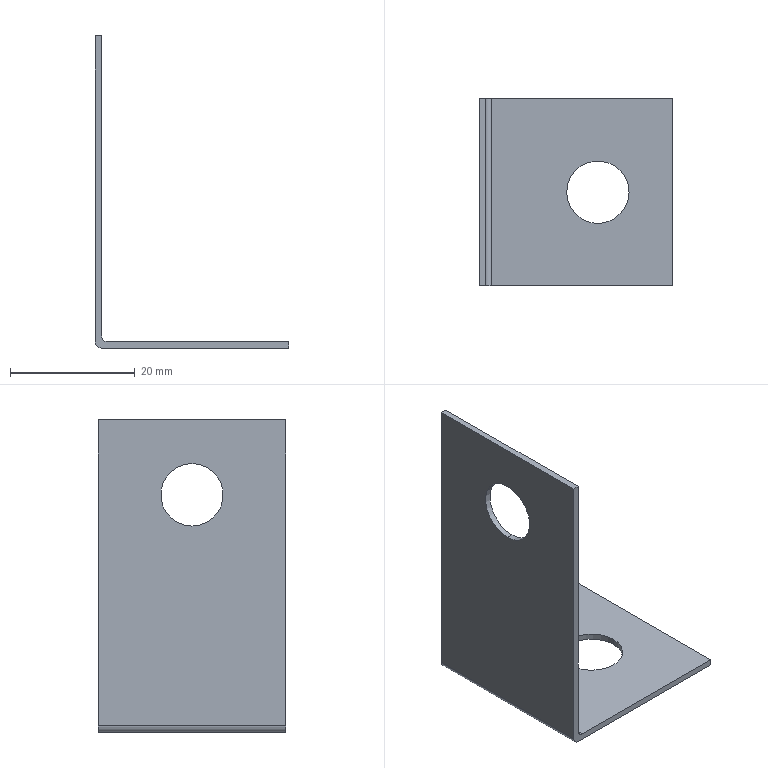Component | SolidWorks | ThreadedConnectionPlate-1 | 1 solid | 14 faces | box 31 x 30 x 50 mm | volume 2243 mm3 | plane 8 | cylinder 6 | commonest cylinder face diameters 10 x4 2 x2
build123d program:
from build123d import *

# Parameters (mm, degrees)
SKETCH1_W           = 30
SKETCH1_H           = 30
BOSS_EXTRUDE1_DEPTH = 1
SKETCH2_W           = 50
SKETCH2_H           = 30
BOSS_EXTRUDE2_DEPTH = 1
FILLET1_R           = 1
SKETCH3_R           = 5
CUT_EXTRUDE1_DEPTH  = 1
SKETCH4_R           = 5
CUT_EXTRUDE2_DEPTH  = 1


with BuildPart() as part:
    # Sketch1 → Boss-Extrude1 (new body)
    with BuildSketch(Plane.XY):
        Rectangle(SKETCH1_W, SKETCH1_H)
    extrude(amount=BOSS_EXTRUDE1_DEPTH)

    # Sketch2 → Boss-Extrude2 (add)
    with BuildSketch(Plane(origin=(15, 0, 0), x_dir=(0, 0, -1), z_dir=(1, 0, 0))):
        with Locations((-25, 0)):
            Rectangle(SKETCH2_W, SKETCH2_H)
    extrude(amount=BOSS_EXTRUDE2_DEPTH)

    # Fillet1
    fillet1_edges = [part.edges().sort_by_distance(p)[0] for p in [
        (16, 0, 0),
        (15, 0, 1),
    ]]
    fillet(fillet1_edges, radius=FILLET1_R)

    # Sketch3 → Cut-Extrude1 (cut)
    with BuildSketch(Plane.XY.offset(1)):
        with Locations((-3, 0)):
            Circle(SKETCH3_R)
    extrude(amount=-CUT_EXTRUDE1_DEPTH, mode=Mode.SUBTRACT)

    # Sketch4 → Cut-Extrude2 (cut)
    with BuildSketch(Plane.ZY.offset(-15)):
        with Locations((38, 0)):
            Circle(SKETCH4_R)
    extrude(amount=-CUT_EXTRUDE2_DEPTH, mode=Mode.SUBTRACT)


solid = part.part

# Placed as in the assembly
solid = solid.moved(Location((102.629, 35.1, 238), (0, 0, 180)))
STEP:
#1=COLOUR_RGB('',0.7922,0.8196,0.9333);
#2=FILL_AREA_STYLE_COLOUR('',#1);
#3=FILL_AREA_STYLE('',(#2));
#4=SURFACE_STYLE_FILL_AREA(#3);
#5=SURFACE_SIDE_STYLE('',(#4));
#6=SURFACE_STYLE_USAGE(.BOTH.,#5);
#7=PRESENTATION_STYLE_ASSIGNMENT((#6));
#8=CARTESIAN_POINT('',(3.411,1.382,10.669));
#9=VERTEX_POINT('',#8);
#10=CARTESIAN_POINT('',(3.411,1.382,11.063));
#11=VERTEX_POINT('',#10);
#12=CARTESIAN_POINT('',(3.411,1.382,10.866));
#13=DIRECTION('',(1.,-0.,0.));
#14=DIRECTION('',(0.,0.,1.));
#15=AXIS2_PLACEMENT_3D('',#12,#13,#14);
#16=CIRCLE('',#15,0.1969);
#17=EDGE_CURVE('',#9,#11,#16,.T.);
#18=ORIENTED_EDGE('',*,*,#17,.F.);
#19=CARTESIAN_POINT('',(3.45,1.382,10.669));
#20=VERTEX_POINT('',#19);
#21=CARTESIAN_POINT('',(3.411,1.382,10.669));
#22=DIRECTION('',(1.,-0.,0.));
#23=VECTOR('',#22,39.37);
#24=LINE('',#21,#23);
#25=EDGE_CURVE('',#9,#20,#24,.T.);
#26=ORIENTED_EDGE('',*,*,#25,.T.);
#27=CARTESIAN_POINT('',(3.45,1.382,11.063));
#28=VERTEX_POINT('',#27);
#29=CARTESIAN_POINT('',(3.45,1.382,10.866));
#30=DIRECTION('',(1.,-0.,0.));
#31=DIRECTION('',(0.,0.,1.));
#32=AXIS2_PLACEMENT_3D('',#29,#30,#31);
#33=CIRCLE('',#32,0.1969);
#34=EDGE_CURVE('',#20,#28,#33,.T.);
#35=ORIENTED_EDGE('',*,*,#34,.T.);
#36=CARTESIAN_POINT('',(3.411,1.382,11.063));
#37=DIRECTION('',(1.,-0.,0.));
#38=VECTOR('',#37,39.37);
#39=LINE('',#36,#38);
#40=EDGE_CURVE('',#11,#28,#39,.T.);
#41=ORIENTED_EDGE('',*,*,#40,.F.);
#42=EDGE_LOOP('',(#18,#26,#35,#41));
#43=FACE_OUTER_BOUND('',#42,.T.);
#44=CARTESIAN_POINT('',(3.411,1.382,10.866));
#45=DIRECTION('',(1.,-0.,0.));
#46=DIRECTION('',(0.,0.,1.));
#47=AXIS2_PLACEMENT_3D('',#44,#45,#46);
#48=CYLINDRICAL_SURFACE('',#47,0.1969);
#49=ADVANCED_FACE('',(#43),#48,.F.);
#50=CARTESIAN_POINT('',(4.355,1.382,9.37));
#51=VERTEX_POINT('',#50);
#52=CARTESIAN_POINT('',(3.962,1.382,9.37));
#53=VERTEX_POINT('',#52);
#54=CARTESIAN_POINT('',(4.159,1.382,9.37));
#55=DIRECTION('',(-0.,0.,1.));
#56=DIRECTION('',(-1.,0.,0.));
#57=AXIS2_PLACEMENT_3D('',#54,#55,#56);
#58=CIRCLE('',#57,0.1969);
#59=EDGE_CURVE('',#51,#53,#58,.T.);
#60=ORIENTED_EDGE('',*,*,#59,.F.);
#61=CARTESIAN_POINT('',(4.355,1.382,9.409));
#62=VERTEX_POINT('',#61);
#63=CARTESIAN_POINT('',(4.355,1.382,9.37));
#64=DIRECTION('',(-0.,0.,1.));
#65=VECTOR('',#64,39.37);
#66=LINE('',#63,#65);
#67=EDGE_CURVE('',#51,#62,#66,.T.);
#68=ORIENTED_EDGE('',*,*,#67,.T.);
#69=CARTESIAN_POINT('',(3.962,1.382,9.409));
#70=VERTEX_POINT('',#69);
#71=CARTESIAN_POINT('',(4.159,1.382,9.409));
#72=DIRECTION('',(-0.,0.,1.));
#73=DIRECTION('',(-1.,0.,0.));
#74=AXIS2_PLACEMENT_3D('',#71,#72,#73);
#75=CIRCLE('',#74,0.1969);
#76=EDGE_CURVE('',#62,#70,#75,.T.);
#77=ORIENTED_EDGE('',*,*,#76,.T.);
#78=CARTESIAN_POINT('',(3.962,1.382,9.37));
#79=DIRECTION('',(-0.,0.,1.));
#80=VECTOR('',#79,39.37);
#81=LINE('',#78,#80);
#82=EDGE_CURVE('',#53,#70,#81,.T.);
#83=ORIENTED_EDGE('',*,*,#82,.F.);
#84=EDGE_LOOP('',(#60,#68,#77,#83));
#85=FACE_OUTER_BOUND('',#84,.T.);
#86=CARTESIAN_POINT('',(4.159,1.382,9.37));
#87=DIRECTION('',(-0.,0.,1.));
#88=DIRECTION('',(-1.,0.,0.));
#89=AXIS2_PLACEMENT_3D('',#86,#87,#88);
#90=CYLINDRICAL_SURFACE('',#89,0.1969);
#91=ADVANCED_FACE('',(#85),#90,.F.);
#92=CARTESIAN_POINT('',(3.411,0.7913,9.409));
#93=VERTEX_POINT('',#92);
#94=CARTESIAN_POINT('',(3.411,0.7913,11.339));
#95=VERTEX_POINT('',#94);
#96=CARTESIAN_POINT('',(3.411,0.7913,9.37));
#97=DIRECTION('',(-0.,0.,1.));
#98=VECTOR('',#97,39.37);
#99=LINE('',#96,#98);
#100=EDGE_CURVE('',#93,#95,#99,.T.);
#101=ORIENTED_EDGE('',*,*,#100,.F.);
#102=CARTESIAN_POINT('',(3.45,0.7913,9.37));
#103=VERTEX_POINT('',#102);
#104=CARTESIAN_POINT('',(3.45,0.7913,9.409));
#105=DIRECTION('',(-0.,-1.,0.));
#106=DIRECTION('',(0.,0.,-1.));
#107=AXIS2_PLACEMENT_3D('',#104,#105,#106);
#108=CIRCLE('',#107,0.03937);
#109=EDGE_CURVE('',#93,#103,#108,.T.);
#110=ORIENTED_EDGE('',*,*,#109,.T.);
#111=CARTESIAN_POINT('',(4.631,0.7913,9.37));
#112=VERTEX_POINT('',#111);
#113=CARTESIAN_POINT('',(4.631,0.7913,9.37));
#114=DIRECTION('',(1.,-0.,0.));
#115=VECTOR('',#114,39.37);
#116=LINE('',#113,#115);
#117=EDGE_CURVE('',#103,#112,#116,.T.);
#118=ORIENTED_EDGE('',*,*,#117,.T.);
#119=CARTESIAN_POINT('',(4.631,0.7913,9.409));
#120=VERTEX_POINT('',#119);
#121=CARTESIAN_POINT('',(4.631,0.7913,9.409));
#122=DIRECTION('',(0.,-0.,-1.));
#123=VECTOR('',#122,39.37);
#124=LINE('',#121,#123);
#125=EDGE_CURVE('',#120,#112,#124,.T.);
#126=ORIENTED_EDGE('',*,*,#125,.F.);
#127=CARTESIAN_POINT('',(3.489,0.7913,9.409));
#128=VERTEX_POINT('',#127);
#129=CARTESIAN_POINT('',(4.631,0.7913,9.409));
#130=DIRECTION('',(1.,-0.,0.));
#131=VECTOR('',#130,39.37);
#132=LINE('',#129,#131);
#133=EDGE_CURVE('',#128,#120,#132,.T.);
#134=ORIENTED_EDGE('',*,*,#133,.F.);
#135=CARTESIAN_POINT('',(3.45,0.7913,9.449));
#136=VERTEX_POINT('',#135);
#137=CARTESIAN_POINT('',(3.489,0.7913,9.449));
#138=DIRECTION('',(0.,1.,-0.));
#139=DIRECTION('',(0.,0.,-1.));
#140=AXIS2_PLACEMENT_3D('',#137,#138,#139);
#141=CIRCLE('',#140,0.03937);
#142=EDGE_CURVE('',#128,#136,#141,.T.);
#143=ORIENTED_EDGE('',*,*,#142,.T.);
#144=CARTESIAN_POINT('',(3.45,0.7913,11.339));
#145=VERTEX_POINT('',#144);
#146=CARTESIAN_POINT('',(3.45,0.7913,9.37));
#147=DIRECTION('',(-0.,0.,1.));
#148=VECTOR('',#147,39.37);
#149=LINE('',#146,#148);
#150=EDGE_CURVE('',#136,#145,#149,.T.);
#151=ORIENTED_EDGE('',*,*,#150,.T.);
#152=CARTESIAN_POINT('',(3.411,0.7913,11.339));
#153=DIRECTION('',(1.,-0.,0.));
#154=VECTOR('',#153,39.37);
#155=LINE('',#152,#154);
#156=EDGE_CURVE('',#95,#145,#155,.T.);
#157=ORIENTED_EDGE('',*,*,#156,.F.);
#158=EDGE_LOOP('',(#101,#110,#118,#126,#134,#143,#151,#157));
#159=FACE_OUTER_BOUND('',#158,.T.);
#160=CARTESIAN_POINT('',(4.631,0.7913,9.409));
#161=DIRECTION('',(0.,1.,-0.));
#162=DIRECTION('',(0.,-0.,-1.));
#163=AXIS2_PLACEMENT_3D('',#160,#161,#162);
#164=PLANE('',#163);
#165=ADVANCED_FACE('',(#159),#164,.F.);
#166=CARTESIAN_POINT('',(4.631,1.972,9.37));
#167=VERTEX_POINT('',#166);
#168=CARTESIAN_POINT('',(4.631,1.972,9.37));
#169=DIRECTION('',(0.,1.,-0.));
#170=VECTOR('',#169,39.37);
#171=LINE('',#168,#170);
#172=EDGE_CURVE('',#112,#167,#171,.T.);
#173=ORIENTED_EDGE('',*,*,#172,.T.);
#174=CARTESIAN_POINT('',(4.631,1.972,9.409));
#175=VERTEX_POINT('',#174);
#176=CARTESIAN_POINT('',(4.631,1.972,9.409));
#177=DIRECTION('',(0.,-0.,-1.));
#178=VECTOR('',#177,39.37);
#179=LINE('',#176,#178);
#180=EDGE_CURVE('',#175,#167,#179,.T.);
#181=ORIENTED_EDGE('',*,*,#180,.F.);
#182=CARTESIAN_POINT('',(4.631,1.972,9.409));
#183=DIRECTION('',(0.,1.,-0.));
#184=VECTOR('',#183,39.37);
#185=LINE('',#182,#184);
#186=EDGE_CURVE('',#120,#175,#185,.T.);
#187=ORIENTED_EDGE('',*,*,#186,.F.);
#188=ORIENTED_EDGE('',*,*,#125,.T.);
#189=EDGE_LOOP('',(#173,#181,#187,#188));
#190=FACE_OUTER_BOUND('',#189,.T.);
#191=CARTESIAN_POINT('',(4.631,1.972,9.409));
#192=DIRECTION('',(-1.,0.,-0.));
#193=DIRECTION('',(0.,-0.,-1.));
#194=AXIS2_PLACEMENT_3D('',#191,#192,#193);
#195=PLANE('',#194);
#196=ADVANCED_FACE('',(#190),#195,.F.);
#197=CARTESIAN_POINT('',(3.45,1.972,9.37));
#198=VERTEX_POINT('',#197);
#199=CARTESIAN_POINT('',(4.631,1.972,9.37));
#200=DIRECTION('',(-1.,0.,-0.));
#201=VECTOR('',#200,39.37);
#202=LINE('',#199,#201);
#203=EDGE_CURVE('',#167,#198,#202,.T.);
#204=ORIENTED_EDGE('',*,*,#203,.T.);
#205=CARTESIAN_POINT('',(3.411,1.972,9.409));
#206=VERTEX_POINT('',#205);
#207=CARTESIAN_POINT('',(3.45,1.972,9.409));
#208=DIRECTION('',(0.,1.,-0.));
#209=DIRECTION('',(0.,0.,1.));
#210=AXIS2_PLACEMENT_3D('',#207,#208,#209);
#211=CIRCLE('',#210,0.03937);
#212=EDGE_CURVE('',#198,#206,#211,.T.);
#213=ORIENTED_EDGE('',*,*,#212,.T.);
#214=CARTESIAN_POINT('',(3.411,1.972,11.339));
#215=VERTEX_POINT('',#214);
#216=CARTESIAN_POINT('',(3.411,1.972,11.339));
#217=DIRECTION('',(0.,-0.,-1.));
#218=VECTOR('',#217,39.37);
#219=LINE('',#216,#218);
#220=EDGE_CURVE('',#215,#206,#219,.T.);
#221=ORIENTED_EDGE('',*,*,#220,.F.);
#222=CARTESIAN_POINT('',(3.45,1.972,11.339));
#223=VERTEX_POINT('',#222);
#224=CARTESIAN_POINT('',(3.411,1.972,11.339));
#225=DIRECTION('',(1.,-0.,0.));
#226=VECTOR('',#225,39.37);
#227=LINE('',#224,#226);
#228=EDGE_CURVE('',#215,#223,#227,.T.);
#229=ORIENTED_EDGE('',*,*,#228,.T.);
#230=CARTESIAN_POINT('',(3.45,1.972,9.449));
#231=VERTEX_POINT('',#230);
#232=CARTESIAN_POINT('',(3.45,1.972,11.339));
#233=DIRECTION('',(0.,-0.,-1.));
#234=VECTOR('',#233,39.37);
#235=LINE('',#232,#234);
#236=EDGE_CURVE('',#223,#231,#235,.T.);
#237=ORIENTED_EDGE('',*,*,#236,.T.);
#238=CARTESIAN_POINT('',(3.489,1.972,9.409));
#239=VERTEX_POINT('',#238);
#240=CARTESIAN_POINT('',(3.489,1.972,9.449));
#241=DIRECTION('',(-0.,-1.,0.));
#242=DIRECTION('',(0.,0.,1.));
#243=AXIS2_PLACEMENT_3D('',#240,#241,#242);
#244=CIRCLE('',#243,0.03937);
#245=EDGE_CURVE('',#231,#239,#244,.T.);
#246=ORIENTED_EDGE('',*,*,#245,.T.);
#247=CARTESIAN_POINT('',(4.631,1.972,9.409));
#248=DIRECTION('',(-1.,0.,-0.));
#249=VECTOR('',#248,39.37);
#250=LINE('',#247,#249);
#251=EDGE_CURVE('',#175,#239,#250,.T.);
#252=ORIENTED_EDGE('',*,*,#251,.F.);
#253=ORIENTED_EDGE('',*,*,#180,.T.);
#254=EDGE_LOOP('',(#204,#213,#221,#229,#237,#246,#252,#253));
#255=FACE_OUTER_BOUND('',#254,.T.);
#256=CARTESIAN_POINT('',(4.631,1.972,9.409));
#257=DIRECTION('',(-0.,-1.,0.));
#258=DIRECTION('',(-0.,0.,1.));
#259=AXIS2_PLACEMENT_3D('',#256,#257,#258);
#260=PLANE('',#259);
#261=ADVANCED_FACE('',(#255),#260,.F.);
#262=CARTESIAN_POINT('',(4.159,1.382,9.409));
#263=DIRECTION('',(-0.,0.,1.));
#264=DIRECTION('',(-1.,0.,0.));
#265=AXIS2_PLACEMENT_3D('',#262,#263,#264);
#266=CIRCLE('',#265,0.1969);
#267=EDGE_CURVE('',#70,#62,#266,.T.);
#268=ORIENTED_EDGE('',*,*,#267,.F.);
#269=ORIENTED_EDGE('',*,*,#76,.F.);
#270=EDGE_LOOP('',(#268,#269));
#271=FACE_BOUND('',#270,.T.);
#272=ORIENTED_EDGE('',*,*,#251,.T.);
#273=CARTESIAN_POINT('',(3.489,0.7913,9.409));
#274=DIRECTION('',(-0.,-1.,0.));
#275=VECTOR('',#274,39.37);
#276=LINE('',#273,#275);
#277=EDGE_CURVE('',#239,#128,#276,.T.);
#278=ORIENTED_EDGE('',*,*,#277,.T.);
#279=ORIENTED_EDGE('',*,*,#133,.T.);
#280=ORIENTED_EDGE('',*,*,#186,.T.);
#281=EDGE_LOOP('',(#272,#278,#279,#280));
#282=FACE_OUTER_BOUND('',#281,.T.);
#283=CARTESIAN_POINT('',(4.041,1.382,9.409));
#284=DIRECTION('',(0.,-0.,-1.));
#285=DIRECTION('',(1.,-0.,0.));
#286=AXIS2_PLACEMENT_3D('',#283,#284,#285);
#287=PLANE('',#286);
#288=ADVANCED_FACE('',(#271,#282),#287,.F.);
#289=CARTESIAN_POINT('',(4.159,1.382,9.37));
#290=DIRECTION('',(-0.,0.,1.));
#291=DIRECTION('',(-1.,0.,0.));
#292=AXIS2_PLACEMENT_3D('',#289,#290,#291);
#293=CIRCLE('',#292,0.1969);
#294=EDGE_CURVE('',#53,#51,#293,.T.);
#295=ORIENTED_EDGE('',*,*,#294,.T.);
#296=ORIENTED_EDGE('',*,*,#59,.T.);
#297=EDGE_LOOP('',(#295,#296));
#298=FACE_BOUND('',#297,.T.);
#299=ORIENTED_EDGE('',*,*,#117,.F.);
#300=CARTESIAN_POINT('',(3.45,1.382,9.37));
#301=DIRECTION('',(0.,1.,-0.));
#302=VECTOR('',#301,39.37);
#303=LINE('',#300,#302);
#304=EDGE_CURVE('',#103,#198,#303,.T.);
#305=ORIENTED_EDGE('',*,*,#304,.T.);
#306=ORIENTED_EDGE('',*,*,#203,.F.);
#307=ORIENTED_EDGE('',*,*,#172,.F.);
#308=EDGE_LOOP('',(#299,#305,#306,#307));
#309=FACE_OUTER_BOUND('',#308,.T.);
#310=CARTESIAN_POINT('',(4.041,1.382,9.37));
#311=DIRECTION('',(0.,-0.,-1.));
#312=DIRECTION('',(1.,-0.,0.));
#313=AXIS2_PLACEMENT_3D('',#310,#311,#312);
#314=PLANE('',#313);
#315=ADVANCED_FACE('',(#298,#309),#314,.T.);
#316=CARTESIAN_POINT('',(3.45,0.7913,11.339));
#317=DIRECTION('',(0.,1.,-0.));
#318=VECTOR('',#317,39.37);
#319=LINE('',#316,#318);
#320=EDGE_CURVE('',#145,#223,#319,.T.);
#321=ORIENTED_EDGE('',*,*,#320,.T.);
#322=ORIENTED_EDGE('',*,*,#228,.F.);
#323=CARTESIAN_POINT('',(3.411,0.7913,11.339));
#324=DIRECTION('',(0.,1.,-0.));
#325=VECTOR('',#324,39.37);
#326=LINE('',#323,#325);
#327=EDGE_CURVE('',#95,#215,#326,.T.);
#328=ORIENTED_EDGE('',*,*,#327,.F.);
#329=ORIENTED_EDGE('',*,*,#156,.T.);
#330=EDGE_LOOP('',(#321,#322,#328,#329));
#331=FACE_OUTER_BOUND('',#330,.T.);
#332=CARTESIAN_POINT('',(3.411,0.7913,11.339));
#333=DIRECTION('',(0.,-0.,-1.));
#334=DIRECTION('',(1.,-0.,0.));
#335=AXIS2_PLACEMENT_3D('',#332,#333,#334);
#336=PLANE('',#335);
#337=ADVANCED_FACE('',(#331),#336,.F.);
#338=CARTESIAN_POINT('',(3.411,1.382,10.866));
#339=DIRECTION('',(1.,-0.,0.));
#340=DIRECTION('',(0.,0.,1.));
#341=AXIS2_PLACEMENT_3D('',#338,#339,#340);
#342=CIRCLE('',#341,0.1969);
#343=EDGE_CURVE('',#11,#9,#342,.T.);
#344=ORIENTED_EDGE('',*,*,#343,.T.);
#345=ORIENTED_EDGE('',*,*,#17,.T.);
#346=EDGE_LOOP('',(#344,#345));
#347=FACE_BOUND('',#346,.T.);
#348=ORIENTED_EDGE('',*,*,#220,.T.);
#349=CARTESIAN_POINT('',(3.411,1.382,9.409));
#350=DIRECTION('',(-0.,-1.,0.));
#351=VECTOR('',#350,39.37);
#352=LINE('',#349,#351);
#353=EDGE_CURVE('',#206,#93,#352,.T.);
#354=ORIENTED_EDGE('',*,*,#353,.T.);
#355=ORIENTED_EDGE('',*,*,#100,.T.);
#356=ORIENTED_EDGE('',*,*,#327,.T.);
#357=EDGE_LOOP('',(#348,#354,#355,#356));
#358=FACE_OUTER_BOUND('',#357,.T.);
#359=CARTESIAN_POINT('',(3.411,1.382,9.37));
#360=DIRECTION('',(-1.,0.,-0.));
#361=DIRECTION('',(0.,-0.,-1.));
#362=AXIS2_PLACEMENT_3D('',#359,#360,#361);
#363=PLANE('',#362);
#364=ADVANCED_FACE('',(#347,#358),#363,.T.);
#365=CARTESIAN_POINT('',(3.45,1.382,10.866));
#366=DIRECTION('',(1.,-0.,0.));
#367=DIRECTION('',(0.,0.,1.));
#368=AXIS2_PLACEMENT_3D('',#365,#366,#367);
#369=CIRCLE('',#368,0.1969);
#370=EDGE_CURVE('',#28,#20,#369,.T.);
#371=ORIENTED_EDGE('',*,*,#370,.F.);
#372=ORIENTED_EDGE('',*,*,#34,.F.);
#373=EDGE_LOOP('',(#371,#372));
#374=FACE_BOUND('',#373,.T.);
#375=ORIENTED_EDGE('',*,*,#150,.F.);
#376=CARTESIAN_POINT('',(3.45,1.972,9.449));
#377=DIRECTION('',(0.,1.,-0.));
#378=VECTOR('',#377,39.37);
#379=LINE('',#376,#378);
#380=EDGE_CURVE('',#136,#231,#379,.T.);
#381=ORIENTED_EDGE('',*,*,#380,.T.);
#382=ORIENTED_EDGE('',*,*,#236,.F.);
#383=ORIENTED_EDGE('',*,*,#320,.F.);
#384=EDGE_LOOP('',(#375,#381,#382,#383));
#385=FACE_OUTER_BOUND('',#384,.T.);
#386=CARTESIAN_POINT('',(3.45,1.382,9.37));
#387=DIRECTION('',(-1.,0.,-0.));
#388=DIRECTION('',(0.,-0.,-1.));
#389=AXIS2_PLACEMENT_3D('',#386,#387,#388);
#390=PLANE('',#389);
#391=ADVANCED_FACE('',(#374,#385),#390,.F.);
#392=ORIENTED_EDGE('',*,*,#212,.F.);
#393=ORIENTED_EDGE('',*,*,#304,.F.);
#394=ORIENTED_EDGE('',*,*,#109,.F.);
#395=ORIENTED_EDGE('',*,*,#353,.F.);
#396=EDGE_LOOP('',(#392,#393,#394,#395));
#397=FACE_OUTER_BOUND('',#396,.T.);
#398=CARTESIAN_POINT('',(3.45,1.382,9.409));
#399=DIRECTION('',(-0.,-1.,0.));
#400=DIRECTION('',(0.,0.,1.));
#401=AXIS2_PLACEMENT_3D('',#398,#399,#400);
#402=CYLINDRICAL_SURFACE('',#401,0.03937);
#403=ADVANCED_FACE('',(#397),#402,.T.);
#404=ORIENTED_EDGE('',*,*,#245,.F.);
#405=ORIENTED_EDGE('',*,*,#380,.F.);
#406=ORIENTED_EDGE('',*,*,#142,.F.);
#407=ORIENTED_EDGE('',*,*,#277,.F.);
#408=EDGE_LOOP('',(#404,#405,#406,#407));
#409=FACE_OUTER_BOUND('',#408,.T.);
#410=CARTESIAN_POINT('',(3.489,1.382,9.449));
#411=DIRECTION('',(0.,1.,-0.));
#412=DIRECTION('',(0.,0.,-1.));
#413=AXIS2_PLACEMENT_3D('',#410,#411,#412);
#414=CYLINDRICAL_SURFACE('',#413,0.03937);
#415=ADVANCED_FACE('',(#409),#414,.F.);
#416=ORIENTED_EDGE('',*,*,#67,.F.);
#417=ORIENTED_EDGE('',*,*,#294,.F.);
#418=ORIENTED_EDGE('',*,*,#82,.T.);
#419=ORIENTED_EDGE('',*,*,#267,.T.);
#420=EDGE_LOOP('',(#416,#417,#418,#419));
#421=FACE_OUTER_BOUND('',#420,.T.);
#422=CARTESIAN_POINT('',(4.159,1.382,9.37));
#423=DIRECTION('',(-0.,0.,1.));
#424=DIRECTION('',(-1.,0.,0.));
#425=AXIS2_PLACEMENT_3D('',#422,#423,#424);
#426=CYLINDRICAL_SURFACE('',#425,0.1969);
#427=ADVANCED_FACE('',(#421),#426,.F.);
#428=ORIENTED_EDGE('',*,*,#25,.F.);
#429=ORIENTED_EDGE('',*,*,#343,.F.);
#430=ORIENTED_EDGE('',*,*,#40,.T.);
#431=ORIENTED_EDGE('',*,*,#370,.T.);
#432=EDGE_LOOP('',(#428,#429,#430,#431));
#433=FACE_OUTER_BOUND('',#432,.T.);
#434=CARTESIAN_POINT('',(3.411,1.382,10.866));
#435=DIRECTION('',(1.,-0.,0.));
#436=DIRECTION('',(0.,0.,1.));
#437=AXIS2_PLACEMENT_3D('',#434,#435,#436);
#438=CYLINDRICAL_SURFACE('',#437,0.1969);
#439=ADVANCED_FACE('',(#433),#438,.F.);
#440=CLOSED_SHELL('',(#49,#91,#165,#196,#261,#288,#315,#337,#364,#391,#403,#415,#427,#439));
#441=MANIFOLD_SOLID_BREP('',#440);
#442=STYLED_ITEM('',(#7),#441);
#443=(LENGTH_UNIT()NAMED_UNIT(*)SI_UNIT($,.METRE.));
#444=LENGTH_MEASURE_WITH_UNIT(LENGTH_MEASURE(0.0254),#443);
#445=DIMENSIONAL_EXPONENTS(1.,0.,0.,0.,0.,0.,0.);
#446=(CONVERSION_BASED_UNIT('',#444)LENGTH_UNIT()NAMED_UNIT(#445));
#447=UNCERTAINTY_MEASURE_WITH_UNIT(LENGTH_MEASURE(0.00001),#446,'','');
#448=(NAMED_UNIT(*)PLANE_ANGLE_UNIT()SI_UNIT($,.RADIAN.));
#449=(NAMED_UNIT(*)SI_UNIT($,.STERADIAN.)SOLID_ANGLE_UNIT());
#450=(GEOMETRIC_REPRESENTATION_CONTEXT(3)GLOBAL_UNCERTAINTY_ASSIGNED_CONTEXT((#447))GLOBAL_UNIT_ASSIGNED_CONTEXT((#446,#448,#449))REPRESENTATION_CONTEXT('',''));
#451=MECHANICAL_DESIGN_GEOMETRIC_PRESENTATION_REPRESENTATION('',(#442),#450);
#452=PRESENTATION_LAYER_ASSIGNMENT('','',(#442));
#453=CARTESIAN_POINT('',(0.,0.,0.));
#454=DIRECTION('',(0.,0.,1.));
#455=DIRECTION('',(1.,0.,0.));
#456=AXIS2_PLACEMENT_3D('',#453,#454,#455);
#457=(LENGTH_UNIT()NAMED_UNIT(*)SI_UNIT($,.METRE.));
#458=LENGTH_MEASURE_WITH_UNIT(LENGTH_MEASURE(0.0254),#457);
#459=DIMENSIONAL_EXPONENTS(1.,0.,0.,0.,0.,0.,0.);
#460=(CONVERSION_BASED_UNIT('',#458)LENGTH_UNIT()NAMED_UNIT(#459));
#461=UNCERTAINTY_MEASURE_WITH_UNIT(LENGTH_MEASURE(0.00001),#460,'','');
#462=(NAMED_UNIT(*)PLANE_ANGLE_UNIT()SI_UNIT($,.RADIAN.));
#463=(NAMED_UNIT(*)SI_UNIT($,.STERADIAN.)SOLID_ANGLE_UNIT());
#464=(GEOMETRIC_REPRESENTATION_CONTEXT(3)GLOBAL_UNCERTAINTY_ASSIGNED_CONTEXT((#461))GLOBAL_UNIT_ASSIGNED_CONTEXT((#460,#462,#463))REPRESENTATION_CONTEXT('',''));
#465=ADVANCED_BREP_SHAPE_REPRESENTATION('',(#441,#456),#464);